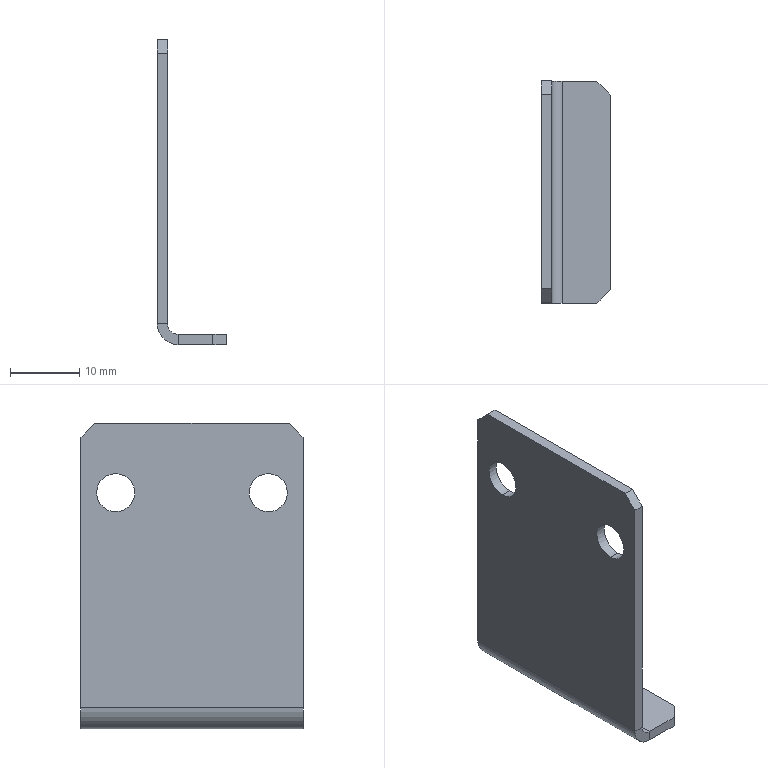Component | SolidWorks | MTCTV2104DJ006-000-0046_SheetMetalPart-1 | 1 solid | 22 faces | box 10 x 32 x 44 mm | volume 2390 mm3 | plane 16 | cylinder 6 | commonest cylinder face diameters 5.5 x4 6 x1 3 x1
STEP:
#1=COLOUR_RGB('',0.7922,0.8196,0.9333);
#2=FILL_AREA_STYLE_COLOUR('',#1);
#3=FILL_AREA_STYLE('',(#2));
#4=SURFACE_STYLE_FILL_AREA(#3);
#5=SURFACE_SIDE_STYLE('',(#4));
#6=SURFACE_STYLE_USAGE(.BOTH.,#5);
#7=PRESENTATION_STYLE_ASSIGNMENT((#6));
#8=CARTESIAN_POINT('',(1.567,1.606,10.559));
#9=VERTEX_POINT('',#8);
#10=CARTESIAN_POINT('',(1.567,1.606,10.342));
#11=VERTEX_POINT('',#10);
#12=CARTESIAN_POINT('',(1.567,1.606,10.451));
#13=DIRECTION('',(1.,0.,0.));
#14=DIRECTION('',(0.,0.,-1.));
#15=AXIS2_PLACEMENT_3D('',#12,#13,#14);
#16=CIRCLE('',#15,0.1083);
#17=EDGE_CURVE('',#9,#11,#16,.T.);
#18=ORIENTED_EDGE('',*,*,#17,.T.);
#19=CARTESIAN_POINT('',(1.508,1.606,10.342));
#20=VERTEX_POINT('',#19);
#21=CARTESIAN_POINT('',(1.508,1.606,10.342));
#22=DIRECTION('',(-1.,-0.,-0.));
#23=VECTOR('',#22,39.37);
#24=LINE('',#21,#23);
#25=EDGE_CURVE('',#11,#20,#24,.T.);
#26=ORIENTED_EDGE('',*,*,#25,.T.);
#27=CARTESIAN_POINT('',(1.508,1.606,10.559));
#28=VERTEX_POINT('',#27);
#29=CARTESIAN_POINT('',(1.508,1.606,10.451));
#30=DIRECTION('',(-1.,-0.,-0.));
#31=DIRECTION('',(0.,0.,1.));
#32=AXIS2_PLACEMENT_3D('',#29,#30,#31);
#33=CIRCLE('',#32,0.1083);
#34=EDGE_CURVE('',#20,#28,#33,.T.);
#35=ORIENTED_EDGE('',*,*,#34,.T.);
#36=CARTESIAN_POINT('',(1.508,1.606,10.559));
#37=DIRECTION('',(-1.,-0.,-0.));
#38=VECTOR('',#37,39.37);
#39=LINE('',#36,#38);
#40=EDGE_CURVE('',#9,#28,#39,.T.);
#41=ORIENTED_EDGE('',*,*,#40,.F.);
#42=EDGE_LOOP('',(#18,#26,#35,#41));
#43=FACE_OUTER_BOUND('',#42,.T.);
#44=CARTESIAN_POINT('',(1.508,1.606,10.451));
#45=DIRECTION('',(-1.,-0.,-0.));
#46=DIRECTION('',(0.,0.,1.));
#47=AXIS2_PLACEMENT_3D('',#44,#45,#46);
#48=CYLINDRICAL_SURFACE('',#47,0.1083);
#49=ADVANCED_FACE('',(#43),#48,.F.);
#50=CARTESIAN_POINT('',(1.567,0.7394,10.559));
#51=VERTEX_POINT('',#50);
#52=CARTESIAN_POINT('',(1.567,0.7394,10.342));
#53=VERTEX_POINT('',#52);
#54=CARTESIAN_POINT('',(1.567,0.7394,10.451));
#55=DIRECTION('',(1.,0.,0.));
#56=DIRECTION('',(0.,0.,-1.));
#57=AXIS2_PLACEMENT_3D('',#54,#55,#56);
#58=CIRCLE('',#57,0.1083);
#59=EDGE_CURVE('',#51,#53,#58,.T.);
#60=ORIENTED_EDGE('',*,*,#59,.T.);
#61=CARTESIAN_POINT('',(1.508,0.7394,10.342));
#62=VERTEX_POINT('',#61);
#63=CARTESIAN_POINT('',(1.508,0.7394,10.342));
#64=DIRECTION('',(-1.,-0.,-0.));
#65=VECTOR('',#64,39.37);
#66=LINE('',#63,#65);
#67=EDGE_CURVE('',#53,#62,#66,.T.);
#68=ORIENTED_EDGE('',*,*,#67,.T.);
#69=CARTESIAN_POINT('',(1.508,0.7394,10.559));
#70=VERTEX_POINT('',#69);
#71=CARTESIAN_POINT('',(1.508,0.7394,10.451));
#72=DIRECTION('',(-1.,-0.,-0.));
#73=DIRECTION('',(0.,0.,1.));
#74=AXIS2_PLACEMENT_3D('',#71,#72,#73);
#75=CIRCLE('',#74,0.1083);
#76=EDGE_CURVE('',#62,#70,#75,.T.);
#77=ORIENTED_EDGE('',*,*,#76,.T.);
#78=CARTESIAN_POINT('',(1.508,0.7394,10.559));
#79=DIRECTION('',(-1.,-0.,-0.));
#80=VECTOR('',#79,39.37);
#81=LINE('',#78,#80);
#82=EDGE_CURVE('',#51,#70,#81,.T.);
#83=ORIENTED_EDGE('',*,*,#82,.F.);
#84=EDGE_LOOP('',(#60,#68,#77,#83));
#85=FACE_OUTER_BOUND('',#84,.T.);
#86=CARTESIAN_POINT('',(1.508,0.7394,10.451));
#87=DIRECTION('',(-1.,-0.,-0.));
#88=DIRECTION('',(0.,0.,1.));
#89=AXIS2_PLACEMENT_3D('',#86,#87,#88);
#90=CYLINDRICAL_SURFACE('',#89,0.1083);
#91=ADVANCED_FACE('',(#85),#90,.F.);
#92=CARTESIAN_POINT('',(1.508,1.802,10.766));
#93=VERTEX_POINT('',#92);
#94=CARTESIAN_POINT('',(1.508,1.802,9.23));
#95=VERTEX_POINT('',#94);
#96=CARTESIAN_POINT('',(1.508,1.802,9.171));
#97=DIRECTION('',(0.,0.,-1.));
#98=VECTOR('',#97,39.37);
#99=LINE('',#96,#98);
#100=EDGE_CURVE('',#93,#95,#99,.T.);
#101=ORIENTED_EDGE('',*,*,#100,.F.);
#102=CARTESIAN_POINT('',(1.567,1.802,10.766));
#103=VERTEX_POINT('',#102);
#104=CARTESIAN_POINT('',(1.567,1.802,10.766));
#105=DIRECTION('',(1.,0.,0.));
#106=VECTOR('',#105,39.37);
#107=LINE('',#104,#106);
#108=EDGE_CURVE('',#93,#103,#107,.T.);
#109=ORIENTED_EDGE('',*,*,#108,.T.);
#110=CARTESIAN_POINT('',(1.567,1.802,9.23));
#111=VERTEX_POINT('',#110);
#112=CARTESIAN_POINT('',(1.567,1.802,9.171));
#113=DIRECTION('',(0.,0.,-1.));
#114=VECTOR('',#113,39.37);
#115=LINE('',#112,#114);
#116=EDGE_CURVE('',#103,#111,#115,.T.);
#117=ORIENTED_EDGE('',*,*,#116,.T.);
#118=CARTESIAN_POINT('',(1.567,1.802,9.23));
#119=DIRECTION('',(-1.,-0.,-0.));
#120=VECTOR('',#119,39.37);
#121=LINE('',#118,#120);
#122=EDGE_CURVE('',#111,#95,#121,.T.);
#123=ORIENTED_EDGE('',*,*,#122,.T.);
#124=EDGE_LOOP('',(#101,#109,#117,#123));
#125=FACE_OUTER_BOUND('',#124,.T.);
#126=CARTESIAN_POINT('',(1.567,1.802,9.171));
#127=DIRECTION('',(-0.,1.,0.));
#128=DIRECTION('',(0.,0.,-1.));
#129=AXIS2_PLACEMENT_3D('',#126,#127,#128);
#130=PLANE('',#129);
#131=ADVANCED_FACE('',(#125),#130,.T.);
#132=ORIENTED_EDGE('',*,*,#17,.F.);
#133=CARTESIAN_POINT('',(1.567,1.606,10.451));
#134=DIRECTION('',(1.,0.,0.));
#135=DIRECTION('',(0.,0.,-1.));
#136=AXIS2_PLACEMENT_3D('',#133,#134,#135);
#137=CIRCLE('',#136,0.1083);
#138=EDGE_CURVE('',#11,#9,#137,.T.);
#139=ORIENTED_EDGE('',*,*,#138,.F.);
#140=EDGE_LOOP('',(#132,#139));
#141=FACE_BOUND('',#140,.T.);
#142=ORIENTED_EDGE('',*,*,#59,.F.);
#143=CARTESIAN_POINT('',(1.567,0.7394,10.451));
#144=DIRECTION('',(1.,0.,0.));
#145=DIRECTION('',(0.,0.,-1.));
#146=AXIS2_PLACEMENT_3D('',#143,#144,#145);
#147=CIRCLE('',#146,0.1083);
#148=EDGE_CURVE('',#53,#51,#147,.T.);
#149=ORIENTED_EDGE('',*,*,#148,.F.);
#150=EDGE_LOOP('',(#142,#149));
#151=FACE_BOUND('',#150,.T.);
#152=ORIENTED_EDGE('',*,*,#116,.F.);
#153=CARTESIAN_POINT('',(1.567,1.724,10.844));
#154=VERTEX_POINT('',#153);
#155=CARTESIAN_POINT('',(1.567,1.866,10.702));
#156=DIRECTION('',(0.,-0.7071,0.7071));
#157=VECTOR('',#156,39.37);
#158=LINE('',#155,#157);
#159=EDGE_CURVE('',#103,#154,#158,.T.);
#160=ORIENTED_EDGE('',*,*,#159,.T.);
#161=CARTESIAN_POINT('',(1.567,0.6213,10.844));
#162=VERTEX_POINT('',#161);
#163=CARTESIAN_POINT('',(1.567,0.5426,10.844));
#164=DIRECTION('',(-0.,1.,0.));
#165=VECTOR('',#164,39.37);
#166=LINE('',#163,#165);
#167=EDGE_CURVE('',#162,#154,#166,.T.);
#168=ORIENTED_EDGE('',*,*,#167,.F.);
#169=CARTESIAN_POINT('',(1.567,0.5426,10.766));
#170=VERTEX_POINT('',#169);
#171=CARTESIAN_POINT('',(1.567,0.4786,10.702));
#172=DIRECTION('',(0.,-0.7071,-0.7071));
#173=VECTOR('',#172,39.37);
#174=LINE('',#171,#173);
#175=EDGE_CURVE('',#162,#170,#174,.T.);
#176=ORIENTED_EDGE('',*,*,#175,.T.);
#177=CARTESIAN_POINT('',(1.567,0.5426,9.23));
#178=VERTEX_POINT('',#177);
#179=CARTESIAN_POINT('',(1.567,0.5426,9.171));
#180=DIRECTION('',(-0.,-0.,1.));
#181=VECTOR('',#180,39.37);
#182=LINE('',#179,#181);
#183=EDGE_CURVE('',#178,#170,#182,.T.);
#184=ORIENTED_EDGE('',*,*,#183,.F.);
#185=CARTESIAN_POINT('',(1.567,1.802,9.23));
#186=DIRECTION('',(0.,-1.,-0.));
#187=VECTOR('',#186,39.37);
#188=LINE('',#185,#187);
#189=EDGE_CURVE('',#111,#178,#188,.T.);
#190=ORIENTED_EDGE('',*,*,#189,.F.);
#191=EDGE_LOOP('',(#152,#160,#168,#176,#184,#190));
#192=FACE_OUTER_BOUND('',#191,.T.);
#193=CARTESIAN_POINT('',(1.567,1.172,10.008));
#194=DIRECTION('',(1.,0.,0.));
#195=DIRECTION('',(0.,0.,-1.));
#196=AXIS2_PLACEMENT_3D('',#193,#194,#195);
#197=PLANE('',#196);
#198=ADVANCED_FACE('',(#141,#151,#192),#197,.T.);
#199=CARTESIAN_POINT('',(1.508,1.606,10.451));
#200=DIRECTION('',(-1.,-0.,-0.));
#201=DIRECTION('',(0.,0.,1.));
#202=AXIS2_PLACEMENT_3D('',#199,#200,#201);
#203=CIRCLE('',#202,0.1083);
#204=EDGE_CURVE('',#28,#20,#203,.T.);
#205=ORIENTED_EDGE('',*,*,#204,.F.);
#206=ORIENTED_EDGE('',*,*,#34,.F.);
#207=EDGE_LOOP('',(#205,#206));
#208=FACE_BOUND('',#207,.T.);
#209=CARTESIAN_POINT('',(1.508,0.7394,10.451));
#210=DIRECTION('',(-1.,-0.,-0.));
#211=DIRECTION('',(0.,0.,1.));
#212=AXIS2_PLACEMENT_3D('',#209,#210,#211);
#213=CIRCLE('',#212,0.1083);
#214=EDGE_CURVE('',#70,#62,#213,.T.);
#215=ORIENTED_EDGE('',*,*,#214,.F.);
#216=ORIENTED_EDGE('',*,*,#76,.F.);
#217=EDGE_LOOP('',(#215,#216));
#218=FACE_BOUND('',#217,.T.);
#219=CARTESIAN_POINT('',(1.508,0.6213,10.844));
#220=VERTEX_POINT('',#219);
#221=CARTESIAN_POINT('',(1.508,1.724,10.844));
#222=VERTEX_POINT('',#221);
#223=CARTESIAN_POINT('',(1.508,0.5426,10.844));
#224=DIRECTION('',(-0.,1.,0.));
#225=VECTOR('',#224,39.37);
#226=LINE('',#223,#225);
#227=EDGE_CURVE('',#220,#222,#226,.T.);
#228=ORIENTED_EDGE('',*,*,#227,.T.);
#229=CARTESIAN_POINT('',(1.508,1.724,10.844));
#230=DIRECTION('',(-0.,0.7071,-0.7071));
#231=VECTOR('',#230,39.37);
#232=LINE('',#229,#231);
#233=EDGE_CURVE('',#222,#93,#232,.T.);
#234=ORIENTED_EDGE('',*,*,#233,.T.);
#235=ORIENTED_EDGE('',*,*,#100,.T.);
#236=CARTESIAN_POINT('',(1.508,0.5426,9.23));
#237=VERTEX_POINT('',#236);
#238=CARTESIAN_POINT('',(1.508,1.802,9.23));
#239=DIRECTION('',(0.,-1.,-0.));
#240=VECTOR('',#239,39.37);
#241=LINE('',#238,#240);
#242=EDGE_CURVE('',#95,#237,#241,.T.);
#243=ORIENTED_EDGE('',*,*,#242,.T.);
#244=CARTESIAN_POINT('',(1.508,0.5426,10.766));
#245=VERTEX_POINT('',#244);
#246=CARTESIAN_POINT('',(1.508,0.5426,9.171));
#247=DIRECTION('',(-0.,-0.,1.));
#248=VECTOR('',#247,39.37);
#249=LINE('',#246,#248);
#250=EDGE_CURVE('',#237,#245,#249,.T.);
#251=ORIENTED_EDGE('',*,*,#250,.T.);
#252=CARTESIAN_POINT('',(1.508,0.5426,10.766));
#253=DIRECTION('',(-0.,0.7071,0.7071));
#254=VECTOR('',#253,39.37);
#255=LINE('',#252,#254);
#256=EDGE_CURVE('',#245,#220,#255,.T.);
#257=ORIENTED_EDGE('',*,*,#256,.T.);
#258=EDGE_LOOP('',(#228,#234,#235,#243,#251,#257));
#259=FACE_OUTER_BOUND('',#258,.T.);
#260=CARTESIAN_POINT('',(1.508,1.172,10.008));
#261=DIRECTION('',(1.,0.,0.));
#262=DIRECTION('',(0.,0.,-1.));
#263=AXIS2_PLACEMENT_3D('',#260,#261,#262);
#264=PLANE('',#263);
#265=ADVANCED_FACE('',(#208,#218,#259),#264,.F.);
#266=ORIENTED_EDGE('',*,*,#167,.T.);
#267=CARTESIAN_POINT('',(1.567,1.724,10.844));
#268=DIRECTION('',(-1.,-0.,-0.));
#269=VECTOR('',#268,39.37);
#270=LINE('',#267,#269);
#271=EDGE_CURVE('',#154,#222,#270,.T.);
#272=ORIENTED_EDGE('',*,*,#271,.T.);
#273=ORIENTED_EDGE('',*,*,#227,.F.);
#274=CARTESIAN_POINT('',(1.567,0.6213,10.844));
#275=DIRECTION('',(1.,0.,0.));
#276=VECTOR('',#275,39.37);
#277=LINE('',#274,#276);
#278=EDGE_CURVE('',#220,#162,#277,.T.);
#279=ORIENTED_EDGE('',*,*,#278,.T.);
#280=EDGE_LOOP('',(#266,#272,#273,#279));
#281=FACE_OUTER_BOUND('',#280,.T.);
#282=CARTESIAN_POINT('',(1.567,0.5426,10.844));
#283=DIRECTION('',(-0.,-0.,1.));
#284=DIRECTION('',(1.,0.,0.));
#285=AXIS2_PLACEMENT_3D('',#282,#283,#284);
#286=PLANE('',#285);
#287=ADVANCED_FACE('',(#281),#286,.T.);
#288=ORIENTED_EDGE('',*,*,#183,.T.);
#289=CARTESIAN_POINT('',(1.567,0.5426,10.766));
#290=DIRECTION('',(-1.,-0.,-0.));
#291=VECTOR('',#290,39.37);
#292=LINE('',#289,#291);
#293=EDGE_CURVE('',#170,#245,#292,.T.);
#294=ORIENTED_EDGE('',*,*,#293,.T.);
#295=ORIENTED_EDGE('',*,*,#250,.F.);
#296=CARTESIAN_POINT('',(1.567,0.5426,9.23));
#297=DIRECTION('',(-1.,-0.,-0.));
#298=VECTOR('',#297,39.37);
#299=LINE('',#296,#298);
#300=EDGE_CURVE('',#178,#237,#299,.T.);
#301=ORIENTED_EDGE('',*,*,#300,.F.);
#302=EDGE_LOOP('',(#288,#294,#295,#301));
#303=FACE_OUTER_BOUND('',#302,.T.);
#304=CARTESIAN_POINT('',(1.567,0.5426,9.171));
#305=DIRECTION('',(0.,-1.,-0.));
#306=DIRECTION('',(-0.,-0.,1.));
#307=AXIS2_PLACEMENT_3D('',#304,#305,#306);
#308=PLANE('',#307);
#309=ADVANCED_FACE('',(#303),#308,.T.);
#310=CARTESIAN_POINT('',(1.626,0.5426,9.171));
#311=VERTEX_POINT('',#310);
#312=CARTESIAN_POINT('',(1.626,0.5426,9.112));
#313=VERTEX_POINT('',#312);
#314=CARTESIAN_POINT('',(1.626,0.5426,9.171));
#315=DIRECTION('',(0.,0.,-1.));
#316=VECTOR('',#315,39.37);
#317=LINE('',#314,#316);
#318=EDGE_CURVE('',#311,#313,#317,.T.);
#319=ORIENTED_EDGE('',*,*,#318,.F.);
#320=CARTESIAN_POINT('',(1.626,0.5426,9.23));
#321=DIRECTION('',(0.,-1.,-0.));
#322=DIRECTION('',(0.,0.,-1.));
#323=AXIS2_PLACEMENT_3D('',#320,#321,#322);
#324=CIRCLE('',#323,0.05906);
#325=EDGE_CURVE('',#178,#311,#324,.T.);
#326=ORIENTED_EDGE('',*,*,#325,.F.);
#327=ORIENTED_EDGE('',*,*,#300,.T.);
#328=CARTESIAN_POINT('',(1.626,0.5426,9.23));
#329=DIRECTION('',(0.,-1.,-0.));
#330=DIRECTION('',(0.,0.,-1.));
#331=AXIS2_PLACEMENT_3D('',#328,#329,#330);
#332=CIRCLE('',#331,0.1181);
#333=EDGE_CURVE('',#237,#313,#332,.T.);
#334=ORIENTED_EDGE('',*,*,#333,.T.);
#335=EDGE_LOOP('',(#319,#326,#327,#334));
#336=FACE_OUTER_BOUND('',#335,.T.);
#337=CARTESIAN_POINT('',(1.626,0.5426,9.23));
#338=DIRECTION('',(0.,-1.,-0.));
#339=DIRECTION('',(-0.,-0.,1.));
#340=AXIS2_PLACEMENT_3D('',#337,#338,#339);
#341=PLANE('',#340);
#342=ADVANCED_FACE('',(#336),#341,.T.);
#343=CARTESIAN_POINT('',(1.626,1.802,9.171));
#344=VERTEX_POINT('',#343);
#345=CARTESIAN_POINT('',(1.626,1.802,9.23));
#346=DIRECTION('',(-0.,1.,0.));
#347=DIRECTION('',(0.,0.,-1.));
#348=AXIS2_PLACEMENT_3D('',#345,#346,#347);
#349=CIRCLE('',#348,0.05906);
#350=EDGE_CURVE('',#344,#111,#349,.T.);
#351=ORIENTED_EDGE('',*,*,#350,.F.);
#352=CARTESIAN_POINT('',(1.626,1.802,9.112));
#353=VERTEX_POINT('',#352);
#354=CARTESIAN_POINT('',(1.626,1.802,9.171));
#355=DIRECTION('',(0.,0.,-1.));
#356=VECTOR('',#355,39.37);
#357=LINE('',#354,#356);
#358=EDGE_CURVE('',#344,#353,#357,.T.);
#359=ORIENTED_EDGE('',*,*,#358,.T.);
#360=CARTESIAN_POINT('',(1.626,1.802,9.23));
#361=DIRECTION('',(-0.,1.,0.));
#362=DIRECTION('',(0.,0.,-1.));
#363=AXIS2_PLACEMENT_3D('',#360,#361,#362);
#364=CIRCLE('',#363,0.1181);
#365=EDGE_CURVE('',#353,#95,#364,.T.);
#366=ORIENTED_EDGE('',*,*,#365,.T.);
#367=ORIENTED_EDGE('',*,*,#122,.F.);
#368=EDGE_LOOP('',(#351,#359,#366,#367));
#369=FACE_OUTER_BOUND('',#368,.T.);
#370=CARTESIAN_POINT('',(1.626,1.802,9.23));
#371=DIRECTION('',(0.,-1.,-0.));
#372=DIRECTION('',(-0.,-0.,1.));
#373=AXIS2_PLACEMENT_3D('',#370,#371,#372);
#374=PLANE('',#373);
#375=ADVANCED_FACE('',(#369),#374,.F.);
#376=ORIENTED_EDGE('',*,*,#242,.F.);
#377=ORIENTED_EDGE('',*,*,#365,.F.);
#378=CARTESIAN_POINT('',(1.626,1.172,9.112));
#379=DIRECTION('',(0.,-1.,-0.));
#380=VECTOR('',#379,39.37);
#381=LINE('',#378,#380);
#382=EDGE_CURVE('',#353,#313,#381,.T.);
#383=ORIENTED_EDGE('',*,*,#382,.T.);
#384=ORIENTED_EDGE('',*,*,#333,.F.);
#385=EDGE_LOOP('',(#376,#377,#383,#384));
#386=FACE_OUTER_BOUND('',#385,.T.);
#387=CARTESIAN_POINT('',(1.626,1.802,9.23));
#388=DIRECTION('',(-0.,1.,0.));
#389=DIRECTION('',(-0.,0.,-1.));
#390=AXIS2_PLACEMENT_3D('',#387,#388,#389);
#391=CYLINDRICAL_SURFACE('',#390,0.1181);
#392=ADVANCED_FACE('',(#386),#391,.T.);
#393=ORIENTED_EDGE('',*,*,#189,.T.);
#394=ORIENTED_EDGE('',*,*,#325,.T.);
#395=CARTESIAN_POINT('',(1.626,0.5426,9.171));
#396=DIRECTION('',(-0.,1.,0.));
#397=VECTOR('',#396,39.37);
#398=LINE('',#395,#397);
#399=EDGE_CURVE('',#311,#344,#398,.T.);
#400=ORIENTED_EDGE('',*,*,#399,.T.);
#401=ORIENTED_EDGE('',*,*,#350,.T.);
#402=EDGE_LOOP('',(#393,#394,#400,#401));
#403=FACE_OUTER_BOUND('',#402,.T.);
#404=CARTESIAN_POINT('',(1.626,1.802,9.23));
#405=DIRECTION('',(-0.,1.,0.));
#406=DIRECTION('',(-0.,0.,-1.));
#407=AXIS2_PLACEMENT_3D('',#404,#405,#406);
#408=CYLINDRICAL_SURFACE('',#407,0.05906);
#409=ADVANCED_FACE('',(#403),#408,.F.);
#410=CARTESIAN_POINT('',(1.823,1.802,9.171));
#411=VERTEX_POINT('',#410);
#412=CARTESIAN_POINT('',(1.902,1.802,9.171));
#413=DIRECTION('',(1.,0.,-0.));
#414=VECTOR('',#413,39.37);
#415=LINE('',#412,#414);
#416=EDGE_CURVE('',#344,#411,#415,.T.);
#417=ORIENTED_EDGE('',*,*,#416,.T.);
#418=CARTESIAN_POINT('',(1.823,1.802,9.112));
#419=VERTEX_POINT('',#418);
#420=CARTESIAN_POINT('',(1.823,1.802,9.112));
#421=DIRECTION('',(-0.,0.,-1.));
#422=VECTOR('',#421,39.37);
#423=LINE('',#420,#422);
#424=EDGE_CURVE('',#411,#419,#423,.T.);
#425=ORIENTED_EDGE('',*,*,#424,.T.);
#426=CARTESIAN_POINT('',(1.902,1.802,9.112));
#427=DIRECTION('',(1.,0.,-0.));
#428=VECTOR('',#427,39.37);
#429=LINE('',#426,#428);
#430=EDGE_CURVE('',#353,#419,#429,.T.);
#431=ORIENTED_EDGE('',*,*,#430,.F.);
#432=ORIENTED_EDGE('',*,*,#358,.F.);
#433=EDGE_LOOP('',(#417,#425,#431,#432));
#434=FACE_OUTER_BOUND('',#433,.T.);
#435=CARTESIAN_POINT('',(1.902,1.802,9.112));
#436=DIRECTION('',(0.,-1.,-0.));
#437=DIRECTION('',(-1.,-0.,-0.));
#438=AXIS2_PLACEMENT_3D('',#435,#436,#437);
#439=PLANE('',#438);
#440=ADVANCED_FACE('',(#434),#439,.F.);
#441=CARTESIAN_POINT('',(1.823,0.5426,9.112));
#442=VERTEX_POINT('',#441);
#443=CARTESIAN_POINT('',(1.567,0.5426,9.112));
#444=DIRECTION('',(-1.,-0.,0.));
#445=VECTOR('',#444,39.37);
#446=LINE('',#443,#445);
#447=EDGE_CURVE('',#442,#313,#446,.T.);
#448=ORIENTED_EDGE('',*,*,#447,.F.);
#449=CARTESIAN_POINT('',(1.823,0.5426,9.171));
#450=VERTEX_POINT('',#449);
#451=CARTESIAN_POINT('',(1.823,0.5426,9.112));
#452=DIRECTION('',(0.,-0.,1.));
#453=VECTOR('',#452,39.37);
#454=LINE('',#451,#453);
#455=EDGE_CURVE('',#442,#450,#454,.T.);
#456=ORIENTED_EDGE('',*,*,#455,.T.);
#457=CARTESIAN_POINT('',(1.567,0.5426,9.171));
#458=DIRECTION('',(-1.,-0.,0.));
#459=VECTOR('',#458,39.37);
#460=LINE('',#457,#459);
#461=EDGE_CURVE('',#450,#311,#460,.T.);
#462=ORIENTED_EDGE('',*,*,#461,.T.);
#463=ORIENTED_EDGE('',*,*,#318,.T.);
#464=EDGE_LOOP('',(#448,#456,#462,#463));
#465=FACE_OUTER_BOUND('',#464,.T.);
#466=CARTESIAN_POINT('',(1.567,0.5426,9.112));
#467=DIRECTION('',(-0.,1.,0.));
#468=DIRECTION('',(1.,0.,0.));
#469=AXIS2_PLACEMENT_3D('',#466,#467,#468);
#470=PLANE('',#469);
#471=ADVANCED_FACE('',(#465),#470,.F.);
#472=ORIENTED_EDGE('',*,*,#430,.T.);
#473=CARTESIAN_POINT('',(1.902,1.724,9.112));
#474=VERTEX_POINT('',#473);
#475=CARTESIAN_POINT('',(1.902,1.724,9.112));
#476=DIRECTION('',(0.7071,-0.7071,-0.));
#477=VECTOR('',#476,39.37);
#478=LINE('',#475,#477);
#479=EDGE_CURVE('',#419,#474,#478,.T.);
#480=ORIENTED_EDGE('',*,*,#479,.T.);
#481=CARTESIAN_POINT('',(1.902,0.6213,9.112));
#482=VERTEX_POINT('',#481);
#483=CARTESIAN_POINT('',(1.902,0.5426,9.112));
#484=DIRECTION('',(0.,-1.,-0.));
#485=VECTOR('',#484,39.37);
#486=LINE('',#483,#485);
#487=EDGE_CURVE('',#474,#482,#486,.T.);
#488=ORIENTED_EDGE('',*,*,#487,.T.);
#489=CARTESIAN_POINT('',(1.823,0.5426,9.112));
#490=DIRECTION('',(-0.7071,-0.7071,0.));
#491=VECTOR('',#490,39.37);
#492=LINE('',#489,#491);
#493=EDGE_CURVE('',#482,#442,#492,.T.);
#494=ORIENTED_EDGE('',*,*,#493,.T.);
#495=ORIENTED_EDGE('',*,*,#447,.T.);
#496=ORIENTED_EDGE('',*,*,#382,.F.);
#497=EDGE_LOOP('',(#472,#480,#488,#494,#495,#496));
#498=FACE_OUTER_BOUND('',#497,.T.);
#499=CARTESIAN_POINT('',(1.508,1.172,9.112));
#500=DIRECTION('',(0.,-0.,1.));
#501=DIRECTION('',(1.,0.,-0.));
#502=AXIS2_PLACEMENT_3D('',#499,#500,#501);
#503=PLANE('',#502);
#504=ADVANCED_FACE('',(#498),#503,.F.);
#505=CARTESIAN_POINT('',(1.902,1.724,9.171));
#506=VERTEX_POINT('',#505);
#507=CARTESIAN_POINT('',(1.902,0.6213,9.171));
#508=VERTEX_POINT('',#507);
#509=CARTESIAN_POINT('',(1.902,0.5426,9.171));
#510=DIRECTION('',(0.,-1.,-0.));
#511=VECTOR('',#510,39.37);
#512=LINE('',#509,#511);
#513=EDGE_CURVE('',#506,#508,#512,.T.);
#514=ORIENTED_EDGE('',*,*,#513,.F.);
#515=CARTESIAN_POINT('',(1.98,1.645,9.171));
#516=DIRECTION('',(-0.7071,0.7071,0.));
#517=VECTOR('',#516,39.37);
#518=LINE('',#515,#517);
#519=EDGE_CURVE('',#506,#411,#518,.T.);
#520=ORIENTED_EDGE('',*,*,#519,.T.);
#521=ORIENTED_EDGE('',*,*,#416,.F.);
#522=ORIENTED_EDGE('',*,*,#399,.F.);
#523=ORIENTED_EDGE('',*,*,#461,.F.);
#524=CARTESIAN_POINT('',(1.98,0.7001,9.171));
#525=DIRECTION('',(0.7071,0.7071,-0.));
#526=VECTOR('',#525,39.37);
#527=LINE('',#524,#526);
#528=EDGE_CURVE('',#450,#508,#527,.T.);
#529=ORIENTED_EDGE('',*,*,#528,.T.);
#530=EDGE_LOOP('',(#514,#520,#521,#522,#523,#529));
#531=FACE_OUTER_BOUND('',#530,.T.);
#532=CARTESIAN_POINT('',(1.508,1.172,9.171));
#533=DIRECTION('',(0.,-0.,1.));
#534=DIRECTION('',(1.,0.,-0.));
#535=AXIS2_PLACEMENT_3D('',#532,#533,#534);
#536=PLANE('',#535);
#537=ADVANCED_FACE('',(#531),#536,.T.);
#538=ORIENTED_EDGE('',*,*,#487,.F.);
#539=CARTESIAN_POINT('',(1.902,1.724,9.112));
#540=DIRECTION('',(0.,-0.,1.));
#541=VECTOR('',#540,39.37);
#542=LINE('',#539,#541);
#543=EDGE_CURVE('',#474,#506,#542,.T.);
#544=ORIENTED_EDGE('',*,*,#543,.T.);
#545=ORIENTED_EDGE('',*,*,#513,.T.);
#546=CARTESIAN_POINT('',(1.902,0.6213,9.112));
#547=DIRECTION('',(-0.,0.,-1.));
#548=VECTOR('',#547,39.37);
#549=LINE('',#546,#548);
#550=EDGE_CURVE('',#508,#482,#549,.T.);
#551=ORIENTED_EDGE('',*,*,#550,.T.);
#552=EDGE_LOOP('',(#538,#544,#545,#551));
#553=FACE_OUTER_BOUND('',#552,.T.);
#554=CARTESIAN_POINT('',(1.902,0.5426,9.112));
#555=DIRECTION('',(-1.,-0.,0.));
#556=DIRECTION('',(0.,-0.,1.));
#557=AXIS2_PLACEMENT_3D('',#554,#555,#556);
#558=PLANE('',#557);
#559=ADVANCED_FACE('',(#553),#558,.F.);
#560=ORIENTED_EDGE('',*,*,#67,.F.);
#561=ORIENTED_EDGE('',*,*,#148,.T.);
#562=ORIENTED_EDGE('',*,*,#82,.T.);
#563=ORIENTED_EDGE('',*,*,#214,.T.);
#564=EDGE_LOOP('',(#560,#561,#562,#563));
#565=FACE_OUTER_BOUND('',#564,.T.);
#566=CARTESIAN_POINT('',(1.508,0.7394,10.451));
#567=DIRECTION('',(-1.,-0.,-0.));
#568=DIRECTION('',(0.,0.,1.));
#569=AXIS2_PLACEMENT_3D('',#566,#567,#568);
#570=CYLINDRICAL_SURFACE('',#569,0.1083);
#571=ADVANCED_FACE('',(#565),#570,.F.);
#572=ORIENTED_EDGE('',*,*,#25,.F.);
#573=ORIENTED_EDGE('',*,*,#138,.T.);
#574=ORIENTED_EDGE('',*,*,#40,.T.);
#575=ORIENTED_EDGE('',*,*,#204,.T.);
#576=EDGE_LOOP('',(#572,#573,#574,#575));
#577=FACE_OUTER_BOUND('',#576,.T.);
#578=CARTESIAN_POINT('',(1.508,1.606,10.451));
#579=DIRECTION('',(-1.,-0.,-0.));
#580=DIRECTION('',(0.,0.,1.));
#581=AXIS2_PLACEMENT_3D('',#578,#579,#580);
#582=CYLINDRICAL_SURFACE('',#581,0.1083);
#583=ADVANCED_FACE('',(#577),#582,.F.);
#584=ORIENTED_EDGE('',*,*,#159,.F.);
#585=ORIENTED_EDGE('',*,*,#108,.F.);
#586=ORIENTED_EDGE('',*,*,#233,.F.);
#587=ORIENTED_EDGE('',*,*,#271,.F.);
#588=EDGE_LOOP('',(#584,#585,#586,#587));
#589=FACE_OUTER_BOUND('',#588,.T.);
#590=CARTESIAN_POINT('',(1.567,1.724,10.844));
#591=DIRECTION('',(0.,-0.7071,-0.7071));
#592=DIRECTION('',(-1.,-0.,-0.));
#593=AXIS2_PLACEMENT_3D('',#590,#591,#592);
#594=PLANE('',#593);
#595=ADVANCED_FACE('',(#589),#594,.F.);
#596=ORIENTED_EDGE('',*,*,#175,.F.);
#597=ORIENTED_EDGE('',*,*,#278,.F.);
#598=ORIENTED_EDGE('',*,*,#256,.F.);
#599=ORIENTED_EDGE('',*,*,#293,.F.);
#600=EDGE_LOOP('',(#596,#597,#598,#599));
#601=FACE_OUTER_BOUND('',#600,.T.);
#602=CARTESIAN_POINT('',(1.567,0.5426,10.766));
#603=DIRECTION('',(-0.,0.7071,-0.7071));
#604=DIRECTION('',(-1.,-0.,-0.));
#605=AXIS2_PLACEMENT_3D('',#602,#603,#604);
#606=PLANE('',#605);
#607=ADVANCED_FACE('',(#601),#606,.F.);
#608=ORIENTED_EDGE('',*,*,#479,.F.);
#609=ORIENTED_EDGE('',*,*,#424,.F.);
#610=ORIENTED_EDGE('',*,*,#519,.F.);
#611=ORIENTED_EDGE('',*,*,#543,.F.);
#612=EDGE_LOOP('',(#608,#609,#610,#611));
#613=FACE_OUTER_BOUND('',#612,.T.);
#614=CARTESIAN_POINT('',(1.902,1.724,9.112));
#615=DIRECTION('',(-0.7071,-0.7071,0.));
#616=DIRECTION('',(0.,-0.,1.));
#617=AXIS2_PLACEMENT_3D('',#614,#615,#616);
#618=PLANE('',#617);
#619=ADVANCED_FACE('',(#613),#618,.F.);
#620=ORIENTED_EDGE('',*,*,#493,.F.);
#621=ORIENTED_EDGE('',*,*,#550,.F.);
#622=ORIENTED_EDGE('',*,*,#528,.F.);
#623=ORIENTED_EDGE('',*,*,#455,.F.);
#624=EDGE_LOOP('',(#620,#621,#622,#623));
#625=FACE_OUTER_BOUND('',#624,.T.);
#626=CARTESIAN_POINT('',(1.823,0.5426,9.112));
#627=DIRECTION('',(-0.7071,0.7071,0.));
#628=DIRECTION('',(0.,-0.,1.));
#629=AXIS2_PLACEMENT_3D('',#626,#627,#628);
#630=PLANE('',#629);
#631=ADVANCED_FACE('',(#625),#630,.F.);
#632=CLOSED_SHELL('',(#49,#91,#131,#198,#265,#287,#309,#342,#375,#392,#409,#440,#471,#504,#537,#559,#571,#583,#595,#607,#619,#631));
#633=MANIFOLD_SOLID_BREP('',#632);
#634=STYLED_ITEM('',(#7),#633);
#635=PRESENTATION_LAYER_ASSIGNMENT('','',(#634));
#636=CARTESIAN_POINT('',(0.,0.,0.));
#637=DIRECTION('',(0.,0.,1.));
#638=DIRECTION('',(1.,0.,0.));
#639=AXIS2_PLACEMENT_3D('',#636,#637,#638);
#640=(LENGTH_UNIT()NAMED_UNIT(*)SI_UNIT($,.METRE.));
#641=LENGTH_MEASURE_WITH_UNIT(LENGTH_MEASURE(0.0254),#640);
#642=DIMENSIONAL_EXPONENTS(1.,0.,0.,0.,0.,0.,0.);
#643=(CONVERSION_BASED_UNIT('',#641)LENGTH_UNIT()NAMED_UNIT(#642));
#644=UNCERTAINTY_MEASURE_WITH_UNIT(LENGTH_MEASURE(0.00001),#643,'','');
#645=(NAMED_UNIT(*)PLANE_ANGLE_UNIT()SI_UNIT($,.RADIAN.));
#646=(NAMED_UNIT(*)SI_UNIT($,.STERADIAN.)SOLID_ANGLE_UNIT());
#647=(GEOMETRIC_REPRESENTATION_CONTEXT(3)GLOBAL_UNCERTAINTY_ASSIGNED_CONTEXT((#644))GLOBAL_UNIT_ASSIGNED_CONTEXT((#643,#645,#646))REPRESENTATION_CONTEXT('',''));
#648=ADVANCED_BREP_SHAPE_REPRESENTATION('',(#633,#639),#647);
#649=(LENGTH_UNIT()NAMED_UNIT(*)SI_UNIT($,.METRE.));
#650=LENGTH_MEASURE_WITH_UNIT(LENGTH_MEASURE(0.0254),#649);
#651=DIMENSIONAL_EXPONENTS(1.,0.,0.,0.,0.,0.,0.);
#652=(CONVERSION_BASED_UNIT('',#650)LENGTH_UNIT()NAMED_UNIT(#651));
#653=UNCERTAINTY_MEASURE_WITH_UNIT(LENGTH_MEASURE(0.00001),#652,'','');
#654=(NAMED_UNIT(*)PLANE_ANGLE_UNIT()SI_UNIT($,.RADIAN.));
#655=(NAMED_UNIT(*)SI_UNIT($,.STERADIAN.)SOLID_ANGLE_UNIT());
#656=(GEOMETRIC_REPRESENTATION_CONTEXT(3)GLOBAL_UNCERTAINTY_ASSIGNED_CONTEXT((#653))GLOBAL_UNIT_ASSIGNED_CONTEXT((#652,#654,#655))REPRESENTATION_CONTEXT('',''));
#657=MECHANICAL_DESIGN_GEOMETRIC_PRESENTATION_REPRESENTATION('',(#634),#656);